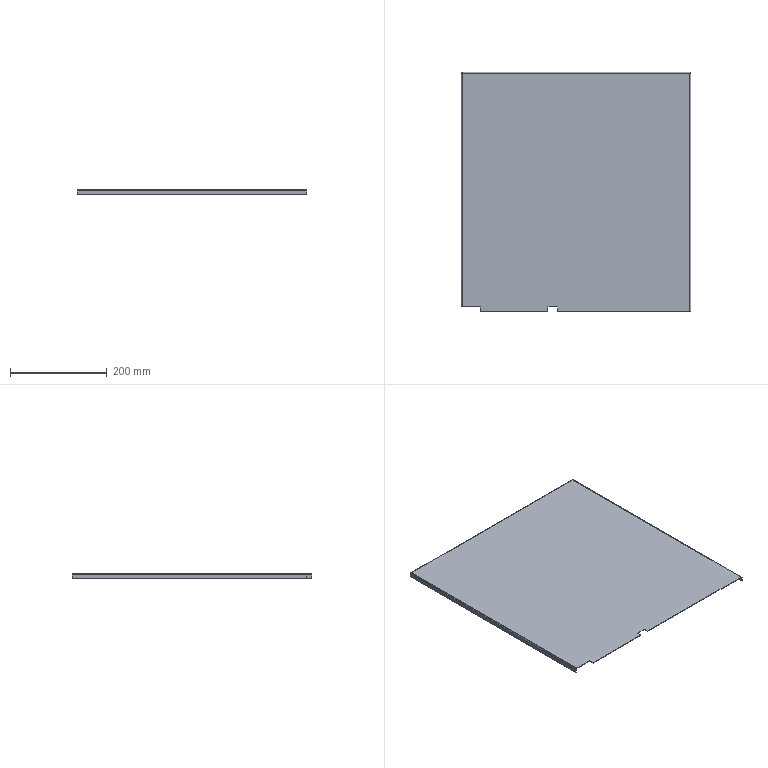Component | SolidWorks | PartitionLeft-1 | 1 solid | 36 faces | volume 296314 mm3 | plane 26 | cylinder 6 | spline 4 | commonest cylinder face diameters 3 x3 5.4 x3